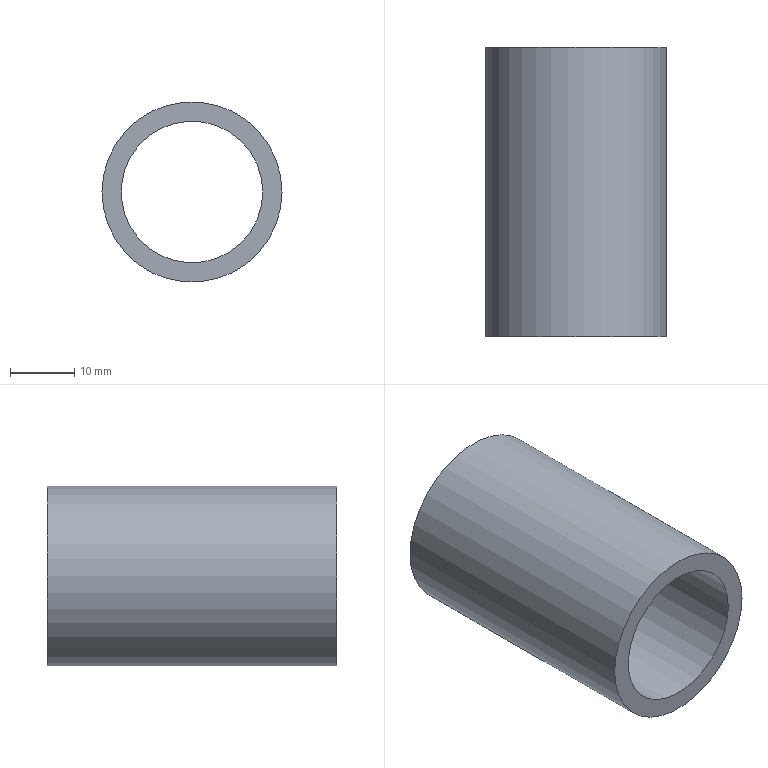Component | NX | BUSHING | 1 solid | 4 faces | box 28 x 45 x 28 mm | volume 10603 mm3 | cylinder 2 | plane 2 | commonest cylinder face diameters 28 x1 22 x1
STEP:
#1=CARTESIAN_POINT('',(0.,0.,0.));
#2=DIRECTION('',(0.,0.,1.));
#3=DIRECTION('',(1.,0.,0.));
#4=AXIS2_PLACEMENT_3D('',#1,#2,#3);
#5=CARTESIAN_POINT('',(14.,19.5,10.75));
#6=VERTEX_POINT('',#5);
#7=CARTESIAN_POINT('',(0.,19.5,10.75));
#8=DIRECTION('',(0.,-1.,0.));
#9=DIRECTION('',(1.,0.,-0.));
#10=AXIS2_PLACEMENT_3D('',#7,#8,#9);
#11=CIRCLE('',#10,14.);
#12=CARTESIAN_POINT('',(0.,19.5,10.75));
#13=DIRECTION('',(0.,-1.,0.));
#14=DIRECTION('',(-1.,0.,0.));
#15=AXIS2_PLACEMENT_3D('',#12,#13,#14);
#16=CYLINDRICAL_SURFACE('',#15,14.);
#17=CARTESIAN_POINT('',(3.142,0.));
#18=DIRECTION('',(1.,0.));
#19=VECTOR('',#18,1.);
#20=LINE('',#17,#19);
#21=(GEOMETRIC_REPRESENTATION_CONTEXT(2)PARAMETRIC_REPRESENTATION_CONTEXT()REPRESENTATION_CONTEXT('',''));
#22=DEFINITIONAL_REPRESENTATION('',(#20),#21);
#23=PCURVE('',#16,#22);
#24=CARTESIAN_POINT('',(0.,19.5,10.75));
#25=DIRECTION('',(0.,-1.,0.));
#26=DIRECTION('',(-1.,0.,0.));
#27=AXIS2_PLACEMENT_3D('',#24,#25,#26);
#28=PLANE('',#27);
#29=CARTESIAN_POINT('',(0.,0.));
#30=DIRECTION('',(-1.,0.));
#31=AXIS2_PLACEMENT_2D('',#29,#30);
#32=CIRCLE('',#31,14.);
#33=(GEOMETRIC_REPRESENTATION_CONTEXT(2)PARAMETRIC_REPRESENTATION_CONTEXT()REPRESENTATION_CONTEXT('',''));
#34=DEFINITIONAL_REPRESENTATION('',(#32),#33);
#35=PCURVE('',#28,#34);
#36=SURFACE_CURVE('',#11,(#23,#35),.PCURVE_S1.);
#37=EDGE_CURVE('',#6,#6,#36,.T.);
#38=ORIENTED_EDGE('',*,*,#37,.T.);
#39=CARTESIAN_POINT('',(14.,-25.5,10.75));
#40=VERTEX_POINT('',#39);
#41=CARTESIAN_POINT('',(14.,19.5,10.75));
#42=CARTESIAN_POINT('',(14.,-25.5,10.75));
#43=B_SPLINE_CURVE_WITH_KNOTS('',1,(#41,#42),.UNSPECIFIED.,.F.,.F.,(2,2),(0.,45.),.PIECEWISE_BEZIER_KNOTS.);
#44=CARTESIAN_POINT('',(9.425,0.));
#45=DIRECTION('',(0.,1.));
#46=VECTOR('',#45,1.);
#47=LINE('',#44,#46);
#48=(GEOMETRIC_REPRESENTATION_CONTEXT(2)PARAMETRIC_REPRESENTATION_CONTEXT()REPRESENTATION_CONTEXT('',''));
#49=DEFINITIONAL_REPRESENTATION('',(#47),#48);
#50=PCURVE('',#16,#49);
#51=CARTESIAN_POINT('',(3.142,0.));
#52=DIRECTION('',(0.,1.));
#53=VECTOR('',#52,1.);
#54=LINE('',#51,#53);
#55=(GEOMETRIC_REPRESENTATION_CONTEXT(2)PARAMETRIC_REPRESENTATION_CONTEXT()REPRESENTATION_CONTEXT('',''));
#56=DEFINITIONAL_REPRESENTATION('',(#54),#55);
#57=PCURVE('',#16,#56);
#58=SEAM_CURVE('',#43,(#50,#57),.PCURVE_S1.);
#59=EDGE_CURVE('',#6,#40,#58,.T.);
#60=ORIENTED_EDGE('',*,*,#59,.T.);
#61=CARTESIAN_POINT('',(0.,-25.5,10.75));
#62=DIRECTION('',(0.,-1.,0.));
#63=DIRECTION('',(1.,0.,-0.));
#64=AXIS2_PLACEMENT_3D('',#61,#62,#63);
#65=CIRCLE('',#64,14.);
#66=CARTESIAN_POINT('',(3.142,45.));
#67=DIRECTION('',(1.,0.));
#68=VECTOR('',#67,1.);
#69=LINE('',#66,#68);
#70=(GEOMETRIC_REPRESENTATION_CONTEXT(2)PARAMETRIC_REPRESENTATION_CONTEXT()REPRESENTATION_CONTEXT('',''));
#71=DEFINITIONAL_REPRESENTATION('',(#69),#70);
#72=PCURVE('',#16,#71);
#73=CARTESIAN_POINT('',(0.,-25.5,10.75));
#74=DIRECTION('',(0.,-1.,0.));
#75=DIRECTION('',(-1.,0.,0.));
#76=AXIS2_PLACEMENT_3D('',#73,#74,#75);
#77=PLANE('',#76);
#78=CARTESIAN_POINT('',(0.,0.));
#79=DIRECTION('',(-1.,0.));
#80=AXIS2_PLACEMENT_2D('',#78,#79);
#81=CIRCLE('',#80,14.);
#82=(GEOMETRIC_REPRESENTATION_CONTEXT(2)PARAMETRIC_REPRESENTATION_CONTEXT()REPRESENTATION_CONTEXT('',''));
#83=DEFINITIONAL_REPRESENTATION('',(#81),#82);
#84=PCURVE('',#77,#83);
#85=SURFACE_CURVE('',#65,(#72,#84),.PCURVE_S1.);
#86=EDGE_CURVE('',#40,#40,#85,.T.);
#87=ORIENTED_EDGE('',*,*,#86,.F.);
#88=ORIENTED_EDGE('',*,*,#59,.F.);
#89=EDGE_LOOP('',(#38,#60,#87,#88));
#90=FACE_BOUND('',#89,.T.);
#91=ADVANCED_FACE('',(#90),#16,.T.);
#92=CARTESIAN_POINT('',(11.,19.5,10.75));
#93=VERTEX_POINT('',#92);
#94=CARTESIAN_POINT('',(0.,19.5,10.75));
#95=DIRECTION('',(0.,-1.,0.));
#96=DIRECTION('',(1.,0.,-0.));
#97=AXIS2_PLACEMENT_3D('',#94,#95,#96);
#98=CIRCLE('',#97,11.);
#99=CARTESIAN_POINT('',(0.,19.5,10.75));
#100=DIRECTION('',(0.,-1.,0.));
#101=DIRECTION('',(-1.,0.,0.));
#102=AXIS2_PLACEMENT_3D('',#99,#100,#101);
#103=CYLINDRICAL_SURFACE('',#102,11.);
#104=CARTESIAN_POINT('',(3.142,0.));
#105=DIRECTION('',(1.,0.));
#106=VECTOR('',#105,1.);
#107=LINE('',#104,#106);
#108=(GEOMETRIC_REPRESENTATION_CONTEXT(2)PARAMETRIC_REPRESENTATION_CONTEXT()REPRESENTATION_CONTEXT('',''));
#109=DEFINITIONAL_REPRESENTATION('',(#107),#108);
#110=PCURVE('',#103,#109);
#111=CARTESIAN_POINT('',(0.,0.));
#112=DIRECTION('',(-1.,0.));
#113=AXIS2_PLACEMENT_2D('',#111,#112);
#114=CIRCLE('',#113,11.);
#115=(GEOMETRIC_REPRESENTATION_CONTEXT(2)PARAMETRIC_REPRESENTATION_CONTEXT()REPRESENTATION_CONTEXT('',''));
#116=DEFINITIONAL_REPRESENTATION('',(#114),#115);
#117=PCURVE('',#28,#116);
#118=SURFACE_CURVE('',#98,(#110,#117),.PCURVE_S1.);
#119=EDGE_CURVE('',#93,#93,#118,.T.);
#120=ORIENTED_EDGE('',*,*,#119,.T.);
#121=CARTESIAN_POINT('',(11.,-25.5,10.75));
#122=VERTEX_POINT('',#121);
#123=CARTESIAN_POINT('',(11.,19.5,10.75));
#124=CARTESIAN_POINT('',(11.,-25.5,10.75));
#125=B_SPLINE_CURVE_WITH_KNOTS('',1,(#123,#124),.UNSPECIFIED.,.F.,.F.,(2,2),(0.,45.),.PIECEWISE_BEZIER_KNOTS.);
#126=CARTESIAN_POINT('',(9.425,0.));
#127=DIRECTION('',(0.,1.));
#128=VECTOR('',#127,1.);
#129=LINE('',#126,#128);
#130=(GEOMETRIC_REPRESENTATION_CONTEXT(2)PARAMETRIC_REPRESENTATION_CONTEXT()REPRESENTATION_CONTEXT('',''));
#131=DEFINITIONAL_REPRESENTATION('',(#129),#130);
#132=PCURVE('',#103,#131);
#133=CARTESIAN_POINT('',(3.142,0.));
#134=DIRECTION('',(0.,1.));
#135=VECTOR('',#134,1.);
#136=LINE('',#133,#135);
#137=(GEOMETRIC_REPRESENTATION_CONTEXT(2)PARAMETRIC_REPRESENTATION_CONTEXT()REPRESENTATION_CONTEXT('',''));
#138=DEFINITIONAL_REPRESENTATION('',(#136),#137);
#139=PCURVE('',#103,#138);
#140=SEAM_CURVE('',#125,(#132,#139),.PCURVE_S1.);
#141=EDGE_CURVE('',#93,#122,#140,.T.);
#142=ORIENTED_EDGE('',*,*,#141,.T.);
#143=CARTESIAN_POINT('',(0.,-25.5,10.75));
#144=DIRECTION('',(0.,-1.,0.));
#145=DIRECTION('',(1.,0.,-0.));
#146=AXIS2_PLACEMENT_3D('',#143,#144,#145);
#147=CIRCLE('',#146,11.);
#148=CARTESIAN_POINT('',(3.142,45.));
#149=DIRECTION('',(1.,0.));
#150=VECTOR('',#149,1.);
#151=LINE('',#148,#150);
#152=(GEOMETRIC_REPRESENTATION_CONTEXT(2)PARAMETRIC_REPRESENTATION_CONTEXT()REPRESENTATION_CONTEXT('',''));
#153=DEFINITIONAL_REPRESENTATION('',(#151),#152);
#154=PCURVE('',#103,#153);
#155=CARTESIAN_POINT('',(0.,0.));
#156=DIRECTION('',(-1.,0.));
#157=AXIS2_PLACEMENT_2D('',#155,#156);
#158=CIRCLE('',#157,11.);
#159=(GEOMETRIC_REPRESENTATION_CONTEXT(2)PARAMETRIC_REPRESENTATION_CONTEXT()REPRESENTATION_CONTEXT('',''));
#160=DEFINITIONAL_REPRESENTATION('',(#158),#159);
#161=PCURVE('',#77,#160);
#162=SURFACE_CURVE('',#147,(#154,#161),.PCURVE_S1.);
#163=EDGE_CURVE('',#122,#122,#162,.T.);
#164=ORIENTED_EDGE('',*,*,#163,.F.);
#165=ORIENTED_EDGE('',*,*,#141,.F.);
#166=EDGE_LOOP('',(#120,#142,#164,#165));
#167=FACE_BOUND('',#166,.F.);
#168=ADVANCED_FACE('',(#167),#103,.F.);
#169=ORIENTED_EDGE('',*,*,#37,.F.);
#170=EDGE_LOOP('',(#169));
#171=FACE_BOUND('',#170,.T.);
#172=ORIENTED_EDGE('',*,*,#119,.T.);
#173=EDGE_LOOP('',(#172));
#174=FACE_BOUND('',#173,.T.);
#175=ADVANCED_FACE('',(#171,#174),#28,.F.);
#176=ORIENTED_EDGE('',*,*,#86,.T.);
#177=EDGE_LOOP('',(#176));
#178=FACE_BOUND('',#177,.T.);
#179=ORIENTED_EDGE('',*,*,#163,.F.);
#180=EDGE_LOOP('',(#179));
#181=FACE_BOUND('',#180,.T.);
#182=ADVANCED_FACE('',(#178,#181),#77,.T.);
#183=CLOSED_SHELL('',(#91,#168,#175,#182));
#184=MANIFOLD_SOLID_BREP('',#183);
#185=(LENGTH_UNIT()NAMED_UNIT(*)SI_UNIT(.MILLI.,.METRE.));
#186=UNCERTAINTY_MEASURE_WITH_UNIT(LENGTH_MEASURE(0.00001),#185,'','');
#187=(NAMED_UNIT(*)PLANE_ANGLE_UNIT()SI_UNIT($,.RADIAN.));
#188=(NAMED_UNIT(*)SI_UNIT($,.STERADIAN.)SOLID_ANGLE_UNIT());
#189=(GEOMETRIC_REPRESENTATION_CONTEXT(3)GLOBAL_UNCERTAINTY_ASSIGNED_CONTEXT((#186))GLOBAL_UNIT_ASSIGNED_CONTEXT((#185,#187,#188))REPRESENTATION_CONTEXT('',''));
#190=ADVANCED_BREP_SHAPE_REPRESENTATION('',(#4,#184),#189);